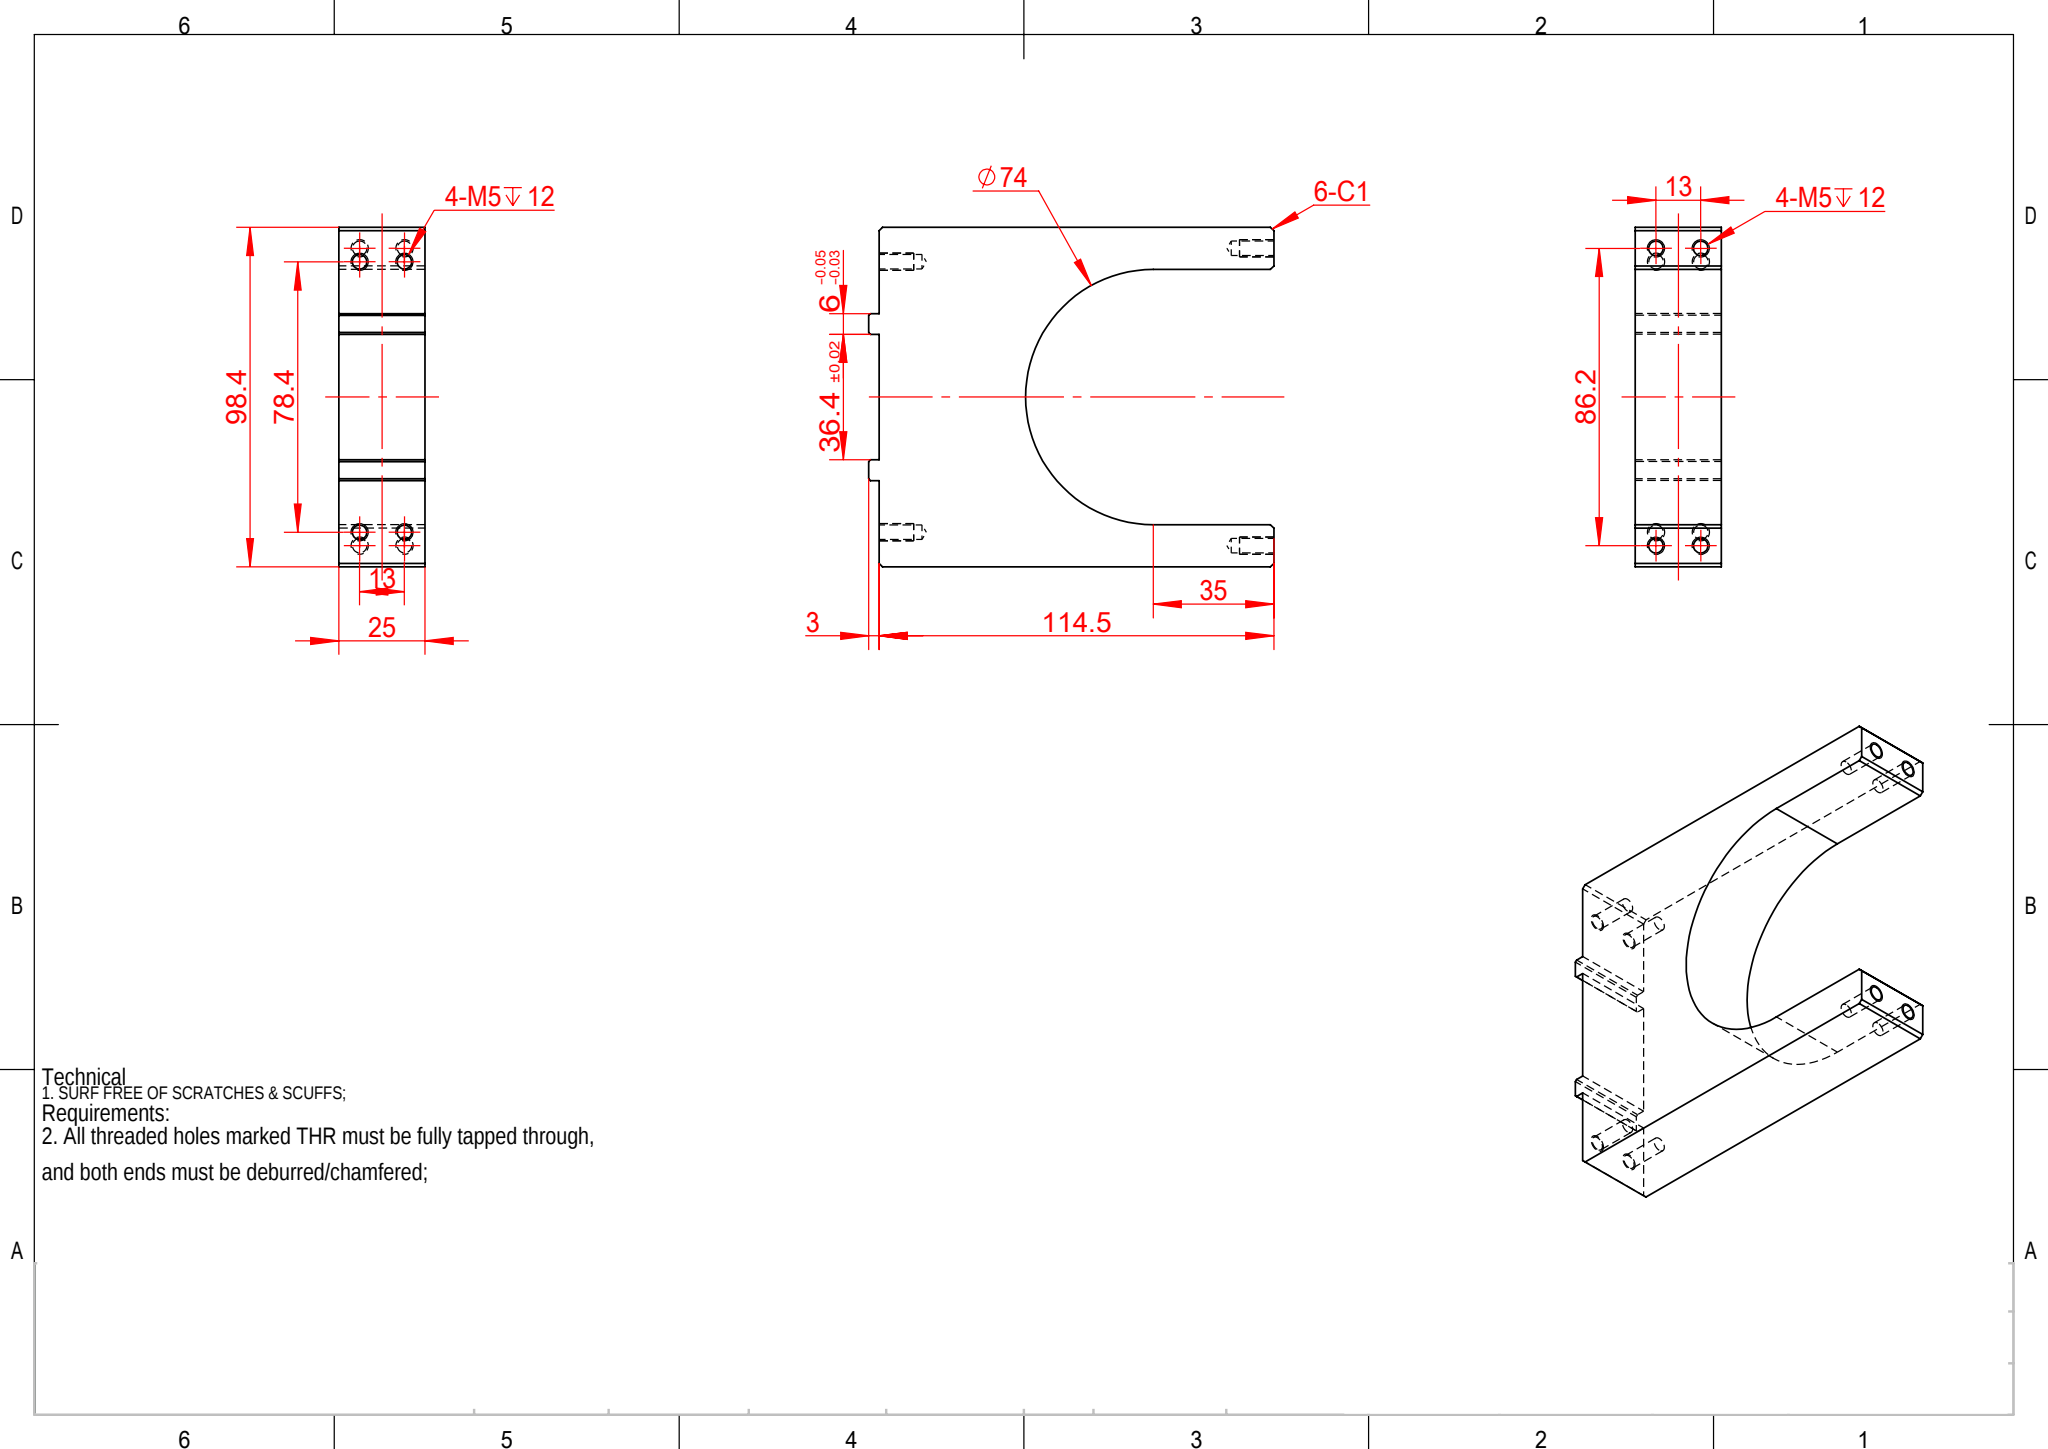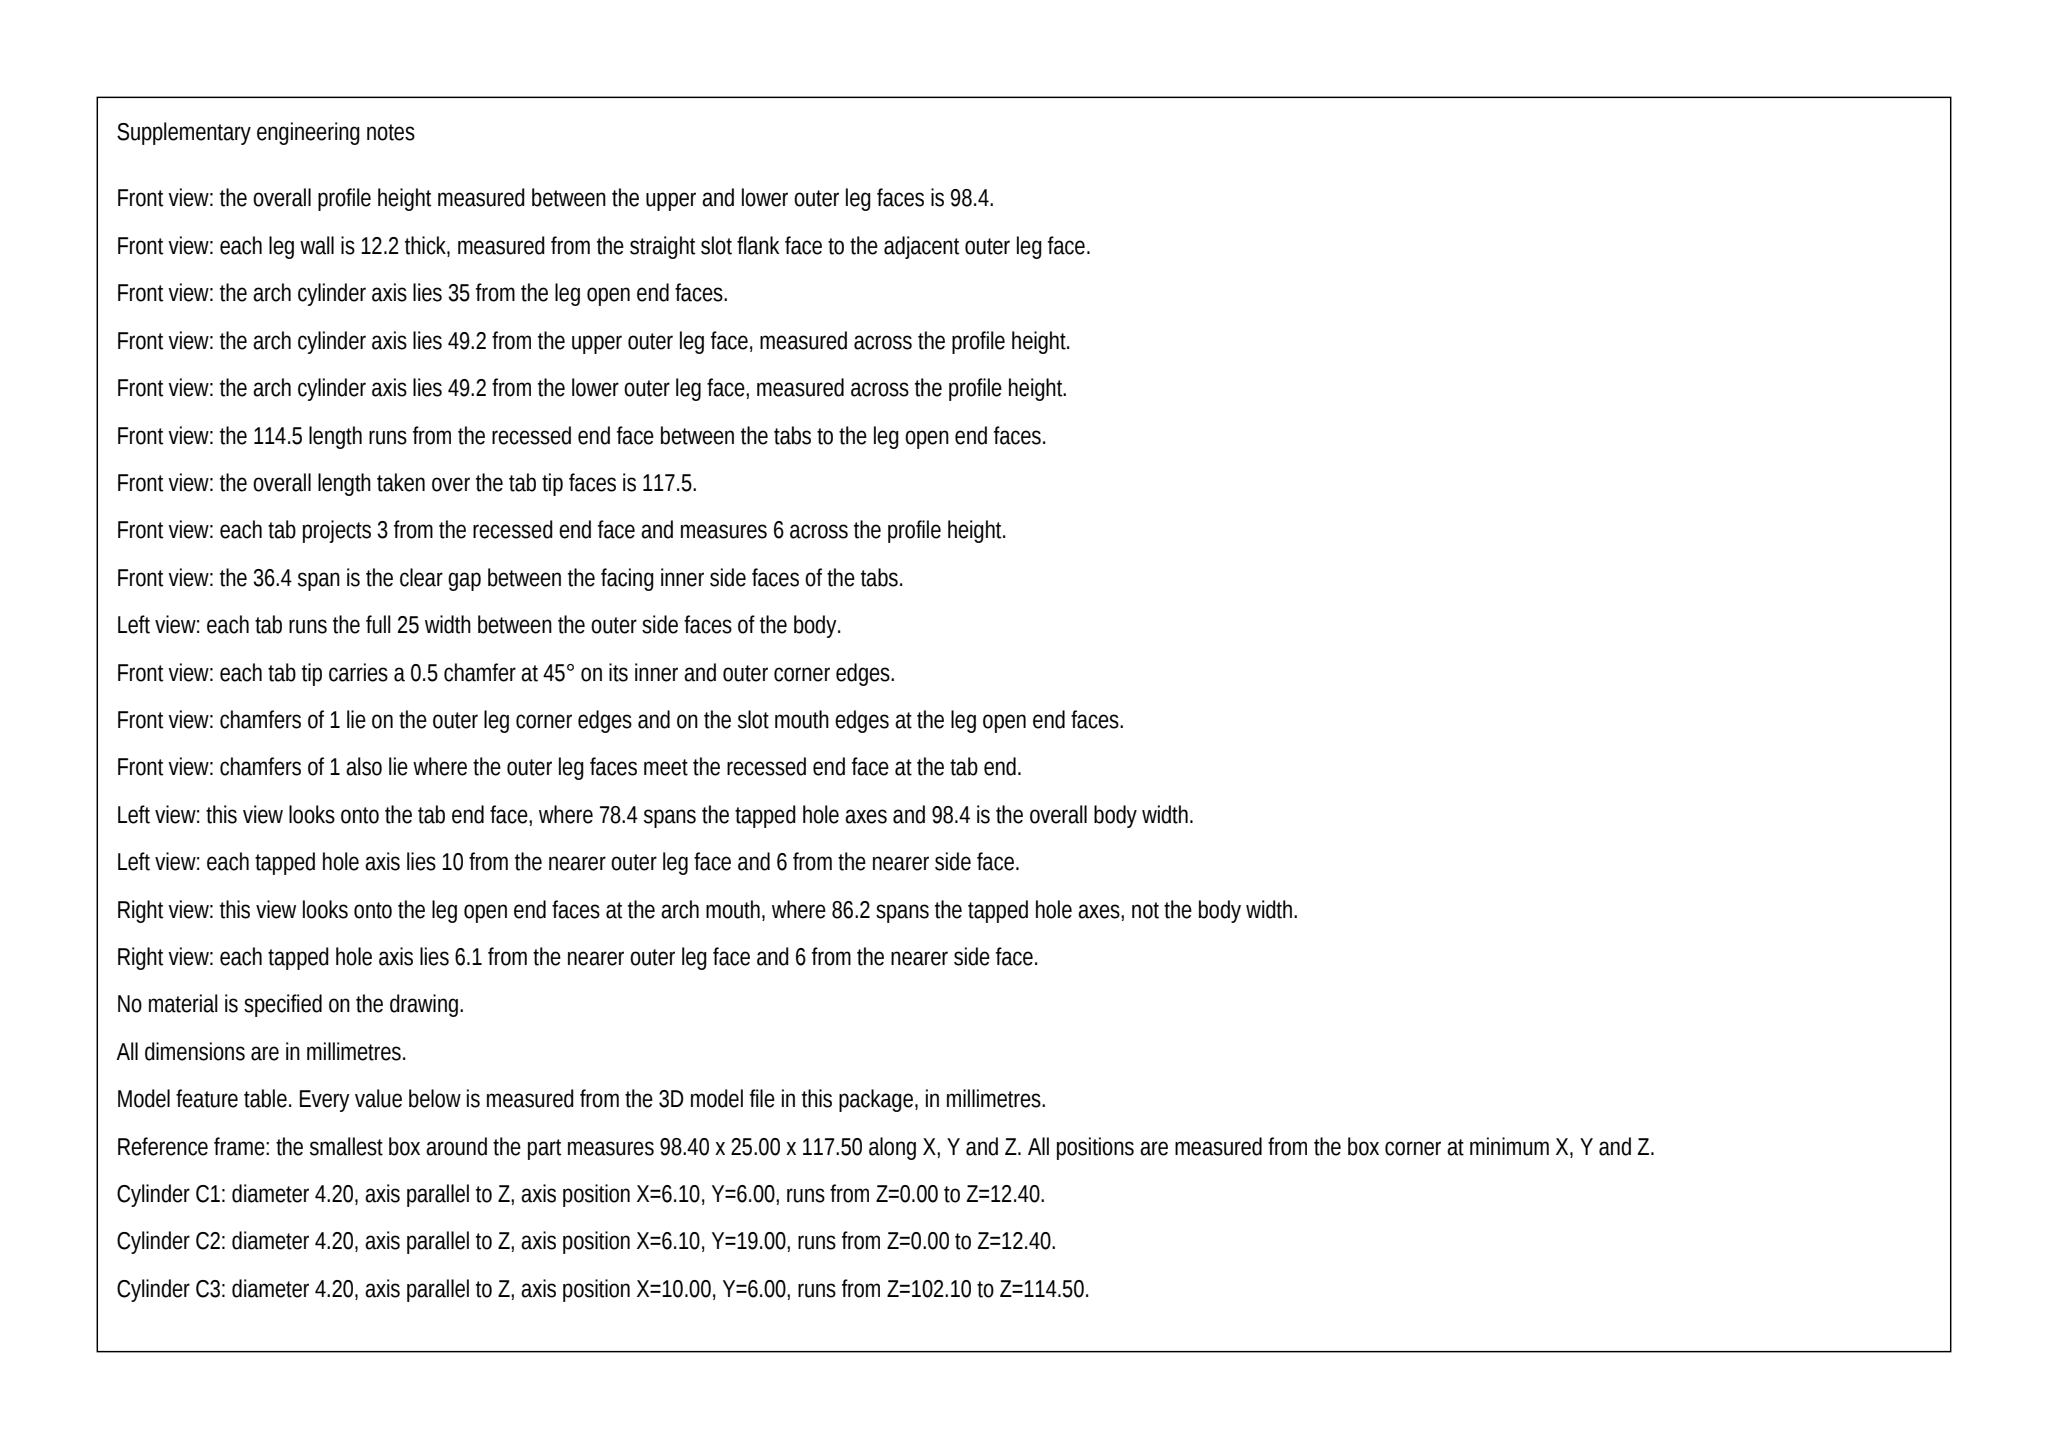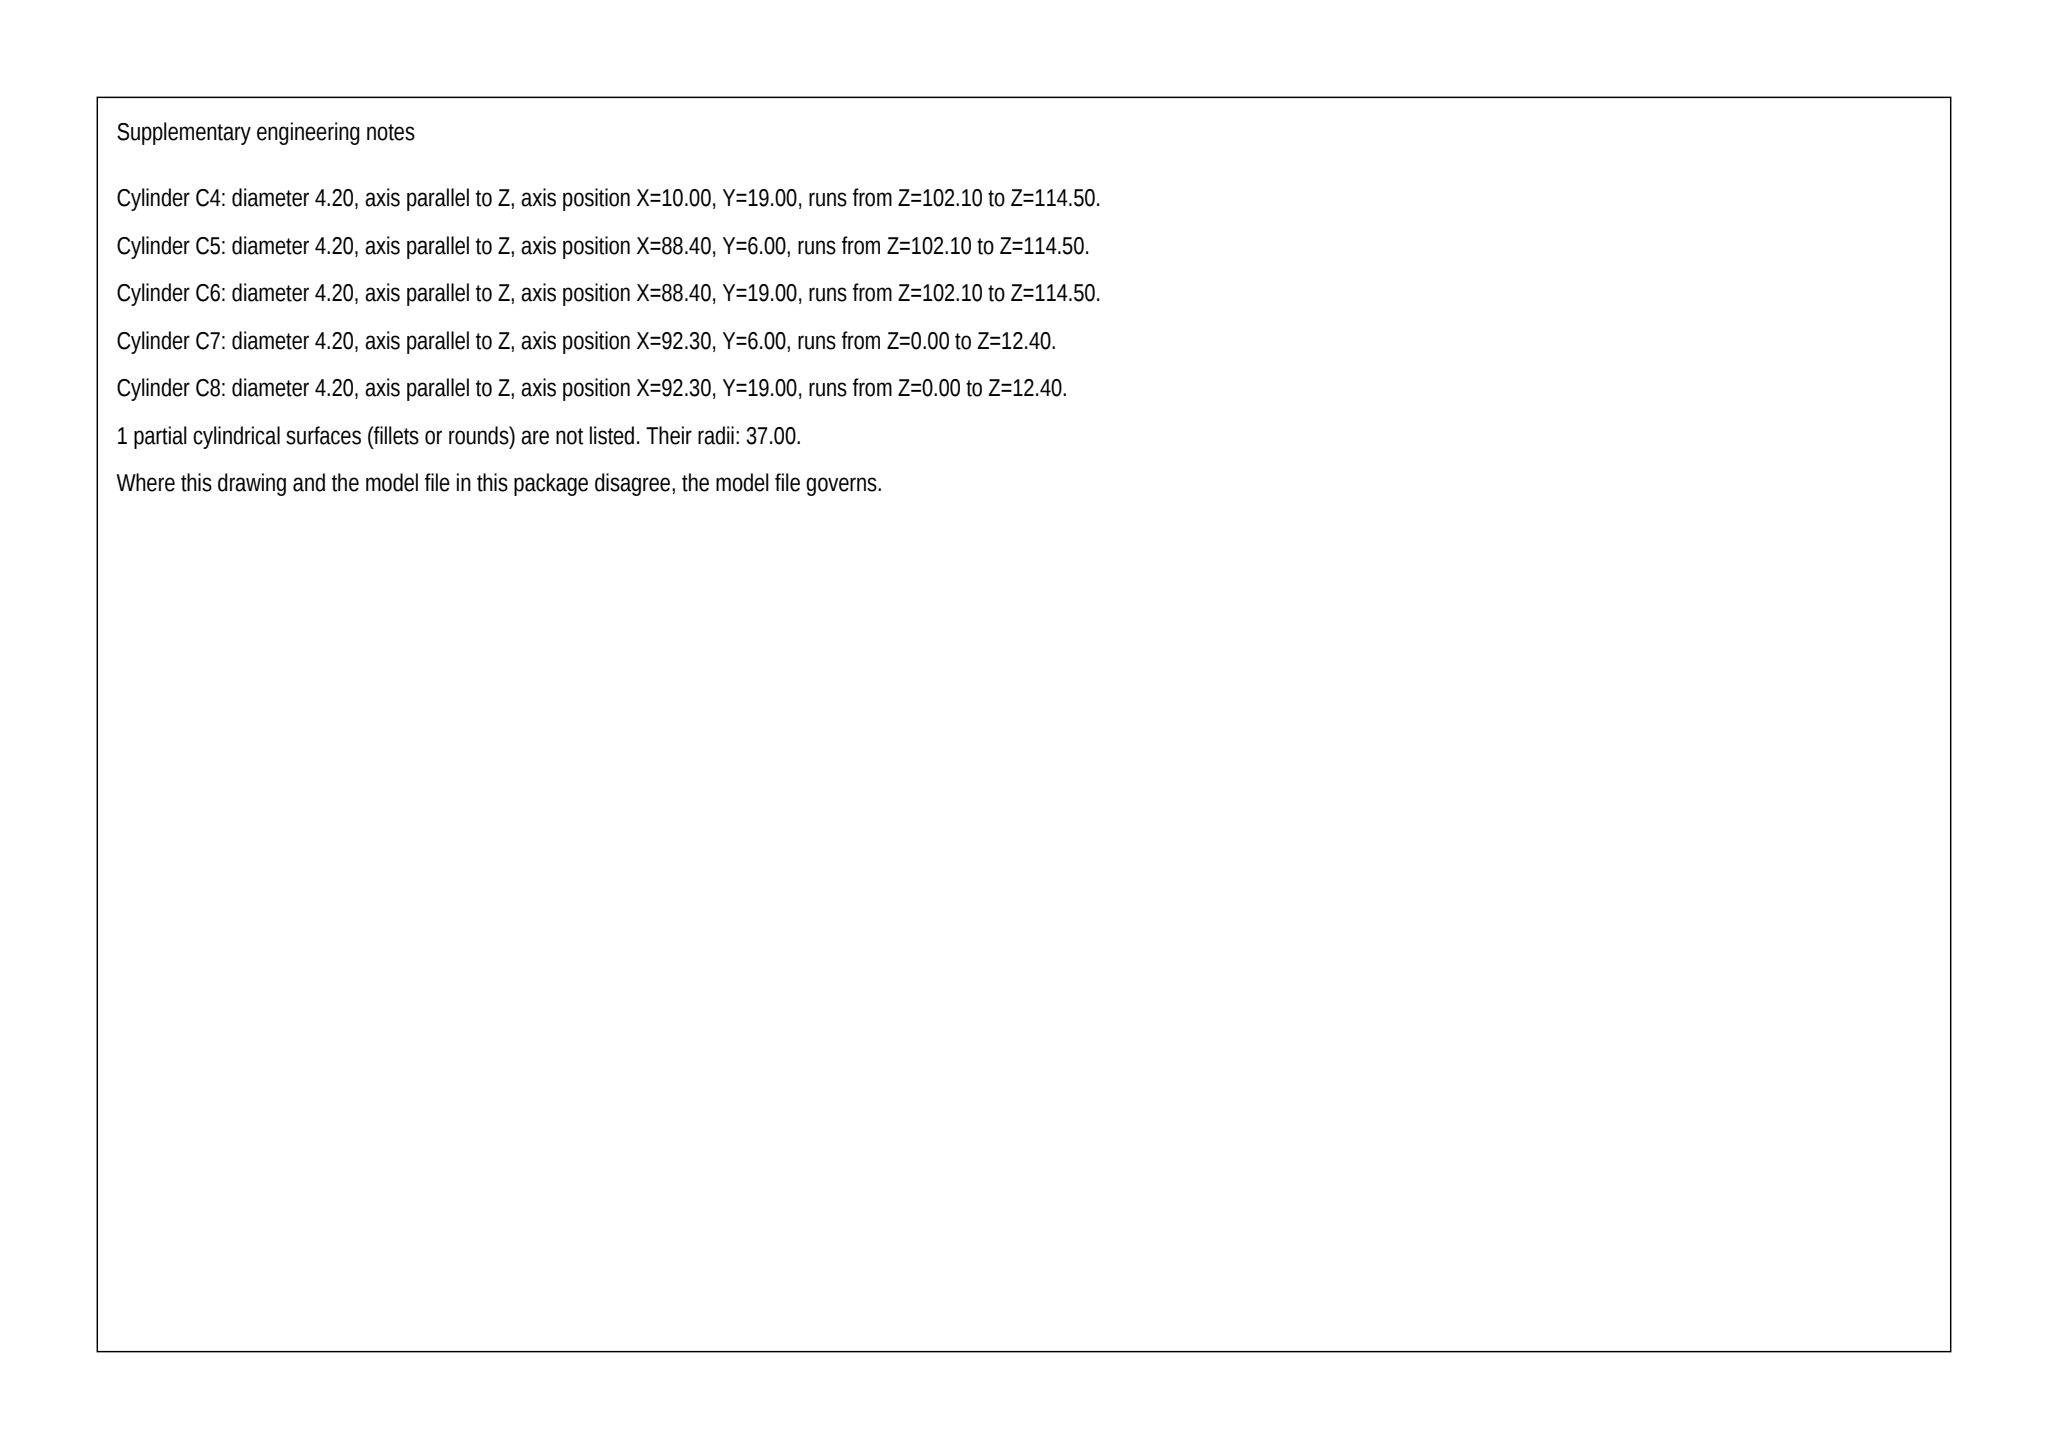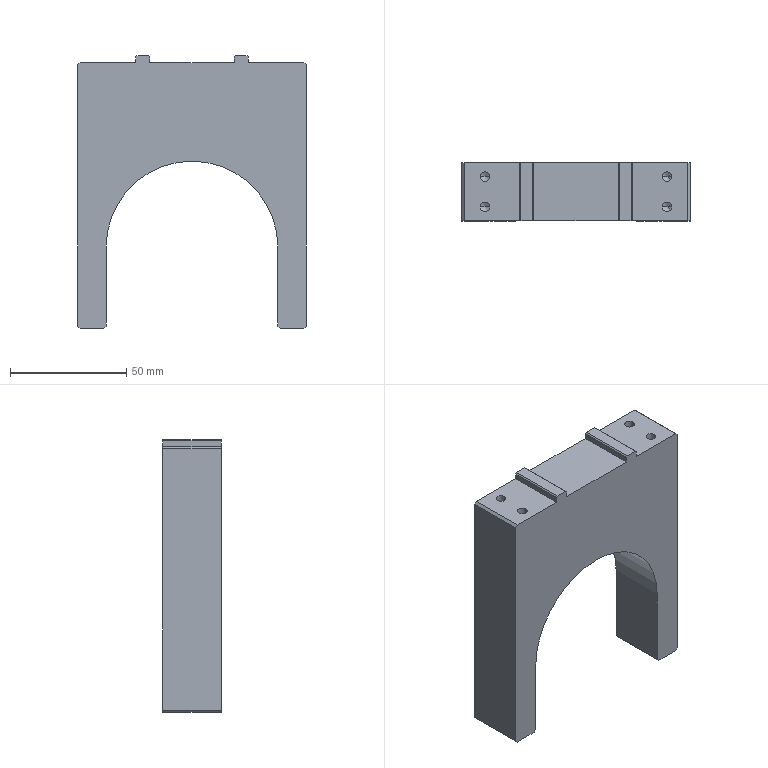Part | SolidWorks | mm | 1 solid | 60 faces | box 98.4 x 25 x 117.5 mm | volume 162551 mm3 | plane 27 | cylinder 17 | cone 16 | commonest cylinder face diameters 4.2 x16 74 x1
Drawing notes:
6 STEP: 6 -0.03/-0.05 (5.97/5.95), 2 PL | from the solid: X planes 25.0-31.0 and 67.4-73.4 give 6.0 nominal step width; 36.4 between 31.0 and 67.4
8-M5 HT 12 EA END FACE (16 TOTAL), WAS 4-M5 HT 12 | from the solid: 16 x Ø4.2 z-axis cylinders, L=12.4, 8 at each z face (z=0 & z=114.5), 118° drill point cones ref Ø4.2 qty 16
M5 HOLE ROWS 6.1 & 10.0 FROM EA END OF 98.4; 13 APART | from the solid: hole x pos 6.1/10.0/88.4/92.3 in 98.4 bbox; y pos 6.0 & 19.0 (13 apart) in 25.0 width
build123d program:
from build123d import *

# Parameters (mm, degrees)
SKETCH1_W                = 98.4
SKETCH1_H                = 25
BOSS_EXTRUDE1_DEPTH      = 114.5
CUT_EXTRUDE2_DEPTH       = 128.106
CUT_EXTRUDE2_DEPTH_BACK  = 128.106
SKETCH6_W                = 6
SKETCH6_H                = 3
BOSS_EXTRUDE2_DEPTH      = 25
CHAMFER1_SIZE            = 0.5
M5_TAPPED_HOLE2_D        = 4.2
M5_TAPPED_HOLE2_DEPTH    = 12.4
M5_TAPPED_HOLE2_TIP      = 1.262
CHAMFER2_SIZE            = 1
CHAMFER1_OF_MIRROR3_SIZE = 0.5


with BuildPart() as part:
    # Sketch1 → Boss-Extrude1 (new body)
    with BuildSketch(Plane.XY):
        Rectangle(SKETCH1_W, SKETCH1_H)
    extrude(amount=BOSS_EXTRUDE1_DEPTH)

    # Sketch3 → Cut-Extrude2 (cut, two sides: drawn at the far end of the back side and taken through both)
    with BuildSketch(Plane(origin=(0, 12.5, 0), x_dir=(1, 0, 0), z_dir=(0, 1, 0)).offset(-CUT_EXTRUDE2_DEPTH_BACK)):
        with BuildLine():
            Line((-37, 296.64), (-37, 0))
            Line((-37, 0), (-37, -35))
            ThreePointArc((-37, -35), (0, -72), (37, -35))
            Line((37, -35), (37, 0))
            Line((37, 0), (37, 296.64))
            Line((37, 296.64), (37, 889.921))
            Line((37, 889.921), (-37, 889.921))
            Line((-37, 889.921), (-37, 296.64))
        make_face()
    extrude(amount=CUT_EXTRUDE2_DEPTH + CUT_EXTRUDE2_DEPTH_BACK, mode=Mode.SUBTRACT)

    # Sketch5 → M5 Tapped Hole1 (revolve, cut)
    with BuildSketch(Plane(origin=(43.1, -6.5, 0), x_dir=(0, 1, 0), z_dir=(1, 0, 0))):
        Polygon((0, 0), (0, 13.662), (2.1, 12.4), (2.1, 0), align=None)
    m5_tapped_hole1 = revolve(axis=Axis((43.1, -6.5, -6.35), (0, 0, 1)), mode=Mode.SUBTRACT)

    # Mirror1: M5 Tapped Hole1 across plane
    add(m5_tapped_hole1.mirror(Plane.ZX), mode=Mode.SUBTRACT)

    # Mirror2: M5 Tapped Hole1 across plane
    add(m5_tapped_hole1.mirror(Plane(origin=(0, 0, 0), x_dir=(0, 0, 1), z_dir=(1, 0, 0))), mode=Mode.SUBTRACT)

    # Mirror2 copy 1 sketch → Mirror2 copy 1 (revolve, cut)
    with BuildSketch(Plane(origin=(-43.1, 6.5, 0), x_dir=(0, -1, 0), z_dir=(-1, 0, 0))):
        Polygon((0, 0), (0, 13.662), (2.1, 12.4), (2.1, 0), align=None)
    revolve(axis=Axis((-43.1, 6.5, -6.35), (0, 0, 1)), mode=Mode.SUBTRACT)

    # Sketch6 → Boss-Extrude2 (add)
    with BuildSketch(Plane(origin=(0, 12.5, 0), x_dir=(1, 0, 0), z_dir=(0, 1, 0))):
        with Locations((21.2, -116)):
            Rectangle(SKETCH6_W, SKETCH6_H)
    boss_extrude2 = extrude(amount=-BOSS_EXTRUDE2_DEPTH)

    # Chamfer1
    chamfer1_edges = [part.edges().sort_by_distance(p)[0] for p in [
        (24.2, 0, 117.5),
        (18.2, 0, 117.5),
    ]]
    chamfer(chamfer1_edges, length=CHAMFER1_SIZE)

    # M5 Tapped Hole2
    with Locations(Plane.XY.offset(114.5)):
        with Locations((-39.2, 6.5), (-39.2, -6.5), (39.2, 6.5), (39.2, -6.5)):
            Hole(M5_TAPPED_HOLE2_D / 2, depth=M5_TAPPED_HOLE2_DEPTH)
            with Locations((0, 0, -(M5_TAPPED_HOLE2_DEPTH + M5_TAPPED_HOLE2_TIP / 2))):  # 118° drill point
                Cone(0, M5_TAPPED_HOLE2_D / 2, M5_TAPPED_HOLE2_TIP, mode=Mode.SUBTRACT)

    # Chamfer2
    chamfer2_edges = [part.edges().sort_by_distance(p)[0] for p in [
        (-49.2, 0, 114.5),
        (37, 0, 0),
        (-37, 0, 0),
        (49.2, 0, 114.5),
        (-49.2, 0, 0),
        (49.2, 0, 0),
    ]]
    chamfer(chamfer2_edges, length=CHAMFER2_SIZE)

    # Mirror3: Boss-Extrude2 across plane
    add(boss_extrude2.mirror(Plane(origin=(0, 0, 0), x_dir=(0, 0, 1), z_dir=(1, 0, 0))))

    # Chamfer1 of Mirror3
    chamfer1_of_mirror3_edges = [part.edges().sort_by_distance(p)[0] for p in [
        (-24.2, 0, 117.5),
        (-18.2, 0, 117.5),
    ]]
    chamfer(chamfer1_of_mirror3_edges, length=CHAMFER1_OF_MIRROR3_SIZE)


solid = part.part